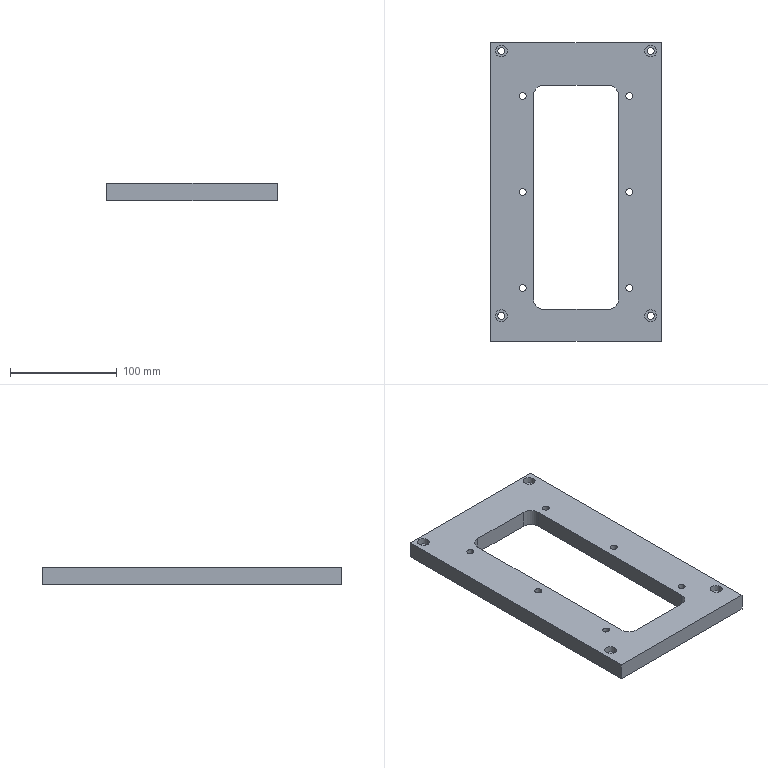Component | NX | BASE | 1 solid | 48 faces | volume 439155 mm3 | cylinder 26 | plane 20 | cone 2 | commonest cylinder face diameters 6.5 x10 11 x10 20 x4 5 x2